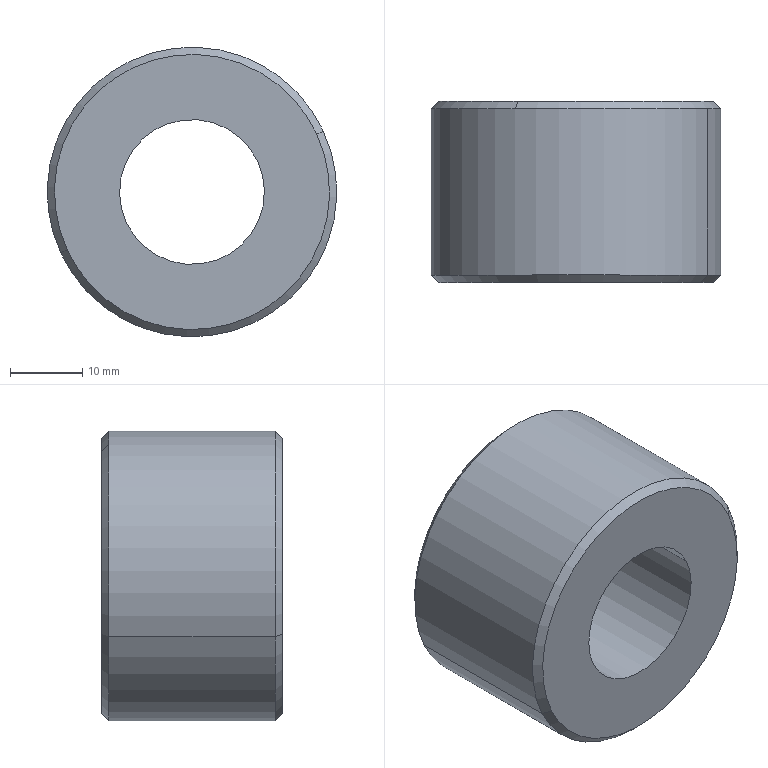Component | SolidWorks | RetainingRing-4 | 1 solid | 10 faces | box 40 x 25 x 40 mm | volume 23438 mm3 | cylinder 4 | cone 4 | plane 2 | commonest cylinder face diameters 20 x2 40 x2
STEP:
#1=CARTESIAN_POINT('',(-9.946,-3.568,-2.197));
#2=VERTEX_POINT('',#1);
#3=CARTESIAN_POINT('',(-10.661,-3.568,-2.528));
#4=VERTEX_POINT('',#3);
#5=CARTESIAN_POINT('',(-10.303,-3.568,-2.362));
#6=DIRECTION('',(-0.,1.,-0.));
#7=DIRECTION('',(-0.9074,0.,-0.4203));
#8=AXIS2_PLACEMENT_3D('',#5,#6,#7);
#9=CIRCLE('',#8,0.3937);
#10=EDGE_CURVE('',#2,#4,#9,.T.);
#11=ORIENTED_EDGE('',*,*,#10,.T.);
#12=CARTESIAN_POINT('',(-10.661,-4.552,-2.528));
#13=VERTEX_POINT('',#12);
#14=CARTESIAN_POINT('',(-10.661,-4.631,-2.528));
#15=DIRECTION('',(0.,-1.,0.));
#16=VECTOR('',#15,39.37);
#17=LINE('',#14,#16);
#18=EDGE_CURVE('',#4,#13,#17,.T.);
#19=ORIENTED_EDGE('',*,*,#18,.T.);
#20=CARTESIAN_POINT('',(-9.946,-4.552,-2.197));
#21=VERTEX_POINT('',#20);
#22=CARTESIAN_POINT('',(-10.303,-4.552,-2.362));
#23=DIRECTION('',(-0.,1.,-0.));
#24=DIRECTION('',(-0.9074,0.,-0.4203));
#25=AXIS2_PLACEMENT_3D('',#22,#23,#24);
#26=CIRCLE('',#25,0.3937);
#27=EDGE_CURVE('',#21,#13,#26,.T.);
#28=ORIENTED_EDGE('',*,*,#27,.F.);
#29=CARTESIAN_POINT('',(-9.946,-4.631,-2.197));
#30=DIRECTION('',(0.,-1.,0.));
#31=VECTOR('',#30,39.37);
#32=LINE('',#29,#31);
#33=EDGE_CURVE('',#2,#21,#32,.T.);
#34=ORIENTED_EDGE('',*,*,#33,.F.);
#35=EDGE_LOOP('',(#11,#19,#28,#34));
#36=FACE_OUTER_BOUND('',#35,.T.);
#37=CARTESIAN_POINT('',(-10.303,-4.631,-2.362));
#38=DIRECTION('',(0.,-1.,0.));
#39=DIRECTION('',(0.9074,0.,0.4203));
#40=AXIS2_PLACEMENT_3D('',#37,#38,#39);
#41=CYLINDRICAL_SURFACE('',#40,0.3937);
#42=ADVANCED_FACE('',(#36),#41,.F.);
#43=CARTESIAN_POINT('',(-10.634,-3.607,-1.648));
#44=VERTEX_POINT('',#43);
#45=CARTESIAN_POINT('',(-11.018,-3.607,-2.693));
#46=VERTEX_POINT('',#45);
#47=CARTESIAN_POINT('',(-10.303,-3.607,-2.362));
#48=DIRECTION('',(0.,-1.,0.));
#49=DIRECTION('',(0.9074,0.,0.4203));
#50=AXIS2_PLACEMENT_3D('',#47,#48,#49);
#51=CIRCLE('',#50,0.7874);
#52=EDGE_CURVE('',#44,#46,#51,.T.);
#53=ORIENTED_EDGE('',*,*,#52,.T.);
#54=CARTESIAN_POINT('',(-11.018,-4.513,-2.693));
#55=VERTEX_POINT('',#54);
#56=CARTESIAN_POINT('',(-11.018,-3.568,-2.693));
#57=DIRECTION('',(0.,-1.,0.));
#58=VECTOR('',#57,39.37);
#59=LINE('',#56,#58);
#60=EDGE_CURVE('',#46,#55,#59,.T.);
#61=ORIENTED_EDGE('',*,*,#60,.T.);
#62=CARTESIAN_POINT('',(-9.589,-4.513,-2.031));
#63=VERTEX_POINT('',#62);
#64=CARTESIAN_POINT('',(-10.303,-4.513,-2.362));
#65=DIRECTION('',(-0.,1.,-0.));
#66=DIRECTION('',(0.9074,0.,0.4203));
#67=AXIS2_PLACEMENT_3D('',#64,#65,#66);
#68=CIRCLE('',#67,0.7874);
#69=EDGE_CURVE('',#55,#63,#68,.T.);
#70=ORIENTED_EDGE('',*,*,#69,.T.);
#71=CARTESIAN_POINT('',(-9.589,-3.607,-2.031));
#72=VERTEX_POINT('',#71);
#73=CARTESIAN_POINT('',(-9.589,-3.568,-2.031));
#74=DIRECTION('',(0.,-1.,0.));
#75=VECTOR('',#74,39.37);
#76=LINE('',#73,#75);
#77=EDGE_CURVE('',#72,#63,#76,.T.);
#78=ORIENTED_EDGE('',*,*,#77,.F.);
#79=CARTESIAN_POINT('',(-10.303,-3.607,-2.362));
#80=DIRECTION('',(0.,-1.,0.));
#81=DIRECTION('',(0.9074,0.,0.4203));
#82=AXIS2_PLACEMENT_3D('',#79,#80,#81);
#83=CIRCLE('',#82,0.7874);
#84=EDGE_CURVE('',#72,#44,#83,.T.);
#85=ORIENTED_EDGE('',*,*,#84,.T.);
#86=EDGE_LOOP('',(#53,#61,#70,#78,#85));
#87=FACE_OUTER_BOUND('',#86,.T.);
#88=CARTESIAN_POINT('',(-10.303,-3.568,-2.362));
#89=DIRECTION('',(0.,-1.,0.));
#90=DIRECTION('',(0.9074,0.,0.4203));
#91=AXIS2_PLACEMENT_3D('',#88,#89,#90);
#92=CYLINDRICAL_SURFACE('',#91,0.7874);
#93=ADVANCED_FACE('',(#87),#92,.T.);
#94=CARTESIAN_POINT('',(-10.982,-4.552,-2.677));
#95=VERTEX_POINT('',#94);
#96=CARTESIAN_POINT('',(-9.625,-4.552,-2.048));
#97=VERTEX_POINT('',#96);
#98=CARTESIAN_POINT('',(-10.303,-4.552,-2.362));
#99=DIRECTION('',(-0.,1.,-0.));
#100=DIRECTION('',(-0.9074,0.,-0.4203));
#101=AXIS2_PLACEMENT_3D('',#98,#99,#100);
#102=CIRCLE('',#101,0.748);
#103=EDGE_CURVE('',#95,#97,#102,.T.);
#104=ORIENTED_EDGE('',*,*,#103,.T.);
#105=CARTESIAN_POINT('',(-9.589,-4.513,-2.031));
#106=DIRECTION('',(0.6416,0.7071,0.2972));
#107=VECTOR('',#106,39.37);
#108=LINE('',#105,#107);
#109=EDGE_CURVE('',#97,#63,#108,.T.);
#110=ORIENTED_EDGE('',*,*,#109,.T.);
#111=ORIENTED_EDGE('',*,*,#69,.F.);
#112=CARTESIAN_POINT('',(-11.018,-4.513,-2.693));
#113=DIRECTION('',(-0.6416,0.7071,-0.2972));
#114=VECTOR('',#113,39.37);
#115=LINE('',#112,#114);
#116=EDGE_CURVE('',#95,#55,#115,.T.);
#117=ORIENTED_EDGE('',*,*,#116,.F.);
#118=EDGE_LOOP('',(#104,#110,#111,#117));
#119=FACE_OUTER_BOUND('',#118,.T.);
#120=CARTESIAN_POINT('',(-10.303,-4.513,-2.362));
#121=DIRECTION('',(-0.,1.,-0.));
#122=DIRECTION('',(-0.9074,0.,-0.4203));
#123=AXIS2_PLACEMENT_3D('',#120,#121,#122);
#124=CONICAL_SURFACE('',#123,0.7874,0.7854);
#125=ADVANCED_FACE('',(#119),#124,.T.);
#126=CARTESIAN_POINT('',(-10.618,-3.568,-1.683));
#127=VERTEX_POINT('',#126);
#128=CARTESIAN_POINT('',(-9.989,-3.568,-3.041));
#129=VERTEX_POINT('',#128);
#130=CARTESIAN_POINT('',(-10.303,-3.568,-2.362));
#131=DIRECTION('',(0.,-1.,0.));
#132=DIRECTION('',(-0.4203,0.,0.9074));
#133=AXIS2_PLACEMENT_3D('',#130,#131,#132);
#134=CIRCLE('',#133,0.748);
#135=EDGE_CURVE('',#127,#129,#134,.T.);
#136=ORIENTED_EDGE('',*,*,#135,.T.);
#137=CARTESIAN_POINT('',(-9.972,-3.607,-3.077));
#138=VERTEX_POINT('',#137);
#139=CARTESIAN_POINT('',(-9.972,-3.607,-3.077));
#140=DIRECTION('',(0.2972,-0.7071,-0.6416));
#141=VECTOR('',#140,39.37);
#142=LINE('',#139,#141);
#143=EDGE_CURVE('',#129,#138,#142,.T.);
#144=ORIENTED_EDGE('',*,*,#143,.T.);
#145=CARTESIAN_POINT('',(-10.303,-3.607,-2.362));
#146=DIRECTION('',(0.,-1.,0.));
#147=DIRECTION('',(0.9074,0.,0.4203));
#148=AXIS2_PLACEMENT_3D('',#145,#146,#147);
#149=CIRCLE('',#148,0.7874);
#150=EDGE_CURVE('',#46,#138,#149,.T.);
#151=ORIENTED_EDGE('',*,*,#150,.F.);
#152=ORIENTED_EDGE('',*,*,#52,.F.);
#153=CARTESIAN_POINT('',(-10.634,-3.607,-1.648));
#154=DIRECTION('',(-0.2972,-0.7071,0.6416));
#155=VECTOR('',#154,39.37);
#156=LINE('',#153,#155);
#157=EDGE_CURVE('',#127,#44,#156,.T.);
#158=ORIENTED_EDGE('',*,*,#157,.F.);
#159=EDGE_LOOP('',(#136,#144,#151,#152,#158));
#160=FACE_OUTER_BOUND('',#159,.T.);
#161=CARTESIAN_POINT('',(-10.303,-3.607,-2.362));
#162=DIRECTION('',(0.,-1.,0.));
#163=DIRECTION('',(-0.4203,0.,0.9074));
#164=AXIS2_PLACEMENT_3D('',#161,#162,#163);
#165=CONICAL_SURFACE('',#164,0.7874,0.7854);
#166=ADVANCED_FACE('',(#160),#165,.T.);
#167=ORIENTED_EDGE('',*,*,#60,.F.);
#168=ORIENTED_EDGE('',*,*,#150,.T.);
#169=CARTESIAN_POINT('',(-10.303,-3.607,-2.362));
#170=DIRECTION('',(0.,-1.,0.));
#171=DIRECTION('',(0.9074,0.,0.4203));
#172=AXIS2_PLACEMENT_3D('',#169,#170,#171);
#173=CIRCLE('',#172,0.7874);
#174=EDGE_CURVE('',#138,#72,#173,.T.);
#175=ORIENTED_EDGE('',*,*,#174,.T.);
#176=ORIENTED_EDGE('',*,*,#77,.T.);
#177=CARTESIAN_POINT('',(-10.303,-4.513,-2.362));
#178=DIRECTION('',(-0.,1.,-0.));
#179=DIRECTION('',(0.9074,0.,0.4203));
#180=AXIS2_PLACEMENT_3D('',#177,#178,#179);
#181=CIRCLE('',#180,0.7874);
#182=EDGE_CURVE('',#63,#55,#181,.T.);
#183=ORIENTED_EDGE('',*,*,#182,.T.);
#184=EDGE_LOOP('',(#167,#168,#175,#176,#183));
#185=FACE_OUTER_BOUND('',#184,.T.);
#186=CARTESIAN_POINT('',(-10.303,-3.568,-2.362));
#187=DIRECTION('',(0.,-1.,0.));
#188=DIRECTION('',(0.9074,0.,0.4203));
#189=AXIS2_PLACEMENT_3D('',#186,#187,#188);
#190=CYLINDRICAL_SURFACE('',#189,0.7874);
#191=ADVANCED_FACE('',(#185),#190,.T.);
#192=ORIENTED_EDGE('',*,*,#109,.F.);
#193=CARTESIAN_POINT('',(-10.303,-4.552,-2.362));
#194=DIRECTION('',(-0.,1.,-0.));
#195=DIRECTION('',(-0.9074,0.,-0.4203));
#196=AXIS2_PLACEMENT_3D('',#193,#194,#195);
#197=CIRCLE('',#196,0.748);
#198=EDGE_CURVE('',#97,#95,#197,.T.);
#199=ORIENTED_EDGE('',*,*,#198,.T.);
#200=ORIENTED_EDGE('',*,*,#116,.T.);
#201=ORIENTED_EDGE('',*,*,#182,.F.);
#202=EDGE_LOOP('',(#192,#199,#200,#201));
#203=FACE_OUTER_BOUND('',#202,.T.);
#204=CARTESIAN_POINT('',(-10.303,-4.513,-2.362));
#205=DIRECTION('',(-0.,1.,-0.));
#206=DIRECTION('',(-0.9074,0.,-0.4203));
#207=AXIS2_PLACEMENT_3D('',#204,#205,#206);
#208=CONICAL_SURFACE('',#207,0.7874,0.7854);
#209=ADVANCED_FACE('',(#203),#208,.T.);
#210=ORIENTED_EDGE('',*,*,#143,.F.);
#211=CARTESIAN_POINT('',(-10.303,-3.568,-2.362));
#212=DIRECTION('',(0.,-1.,0.));
#213=DIRECTION('',(-0.4203,0.,0.9074));
#214=AXIS2_PLACEMENT_3D('',#211,#212,#213);
#215=CIRCLE('',#214,0.748);
#216=EDGE_CURVE('',#129,#127,#215,.T.);
#217=ORIENTED_EDGE('',*,*,#216,.T.);
#218=ORIENTED_EDGE('',*,*,#157,.T.);
#219=ORIENTED_EDGE('',*,*,#84,.F.);
#220=ORIENTED_EDGE('',*,*,#174,.F.);
#221=EDGE_LOOP('',(#210,#217,#218,#219,#220));
#222=FACE_OUTER_BOUND('',#221,.T.);
#223=CARTESIAN_POINT('',(-10.303,-3.607,-2.362));
#224=DIRECTION('',(0.,-1.,0.));
#225=DIRECTION('',(-0.4203,0.,0.9074));
#226=AXIS2_PLACEMENT_3D('',#223,#224,#225);
#227=CONICAL_SURFACE('',#226,0.7874,0.7854);
#228=ADVANCED_FACE('',(#222),#227,.T.);
#229=ORIENTED_EDGE('',*,*,#27,.T.);
#230=CARTESIAN_POINT('',(-10.303,-4.552,-2.362));
#231=DIRECTION('',(-0.,1.,-0.));
#232=DIRECTION('',(-0.9074,0.,-0.4203));
#233=AXIS2_PLACEMENT_3D('',#230,#231,#232);
#234=CIRCLE('',#233,0.3937);
#235=EDGE_CURVE('',#13,#21,#234,.T.);
#236=ORIENTED_EDGE('',*,*,#235,.T.);
#237=EDGE_LOOP('',(#229,#236));
#238=FACE_BOUND('',#237,.T.);
#239=ORIENTED_EDGE('',*,*,#103,.F.);
#240=ORIENTED_EDGE('',*,*,#198,.F.);
#241=EDGE_LOOP('',(#239,#240));
#242=FACE_OUTER_BOUND('',#241,.T.);
#243=CARTESIAN_POINT('',(-10.303,-4.552,-2.362));
#244=DIRECTION('',(-0.,1.,-0.));
#245=DIRECTION('',(-0.9074,-0.,-0.4203));
#246=AXIS2_PLACEMENT_3D('',#243,#244,#245);
#247=PLANE('',#246);
#248=ADVANCED_FACE('',(#238,#242),#247,.F.);
#249=ORIENTED_EDGE('',*,*,#10,.F.);
#250=CARTESIAN_POINT('',(-10.303,-3.568,-2.362));
#251=DIRECTION('',(-0.,1.,-0.));
#252=DIRECTION('',(-0.9074,0.,-0.4203));
#253=AXIS2_PLACEMENT_3D('',#250,#251,#252);
#254=CIRCLE('',#253,0.3937);
#255=EDGE_CURVE('',#4,#2,#254,.T.);
#256=ORIENTED_EDGE('',*,*,#255,.F.);
#257=EDGE_LOOP('',(#249,#256));
#258=FACE_BOUND('',#257,.T.);
#259=ORIENTED_EDGE('',*,*,#135,.F.);
#260=ORIENTED_EDGE('',*,*,#216,.F.);
#261=EDGE_LOOP('',(#259,#260));
#262=FACE_OUTER_BOUND('',#261,.T.);
#263=CARTESIAN_POINT('',(-10.303,-3.568,-2.362));
#264=DIRECTION('',(-0.,1.,-0.));
#265=DIRECTION('',(-0.9074,-0.,-0.4203));
#266=AXIS2_PLACEMENT_3D('',#263,#264,#265);
#267=PLANE('',#266);
#268=ADVANCED_FACE('',(#258,#262),#267,.T.);
#269=ORIENTED_EDGE('',*,*,#18,.F.);
#270=ORIENTED_EDGE('',*,*,#255,.T.);
#271=ORIENTED_EDGE('',*,*,#33,.T.);
#272=ORIENTED_EDGE('',*,*,#235,.F.);
#273=EDGE_LOOP('',(#269,#270,#271,#272));
#274=FACE_OUTER_BOUND('',#273,.T.);
#275=CARTESIAN_POINT('',(-10.303,-4.631,-2.362));
#276=DIRECTION('',(0.,-1.,0.));
#277=DIRECTION('',(0.9074,0.,0.4203));
#278=AXIS2_PLACEMENT_3D('',#275,#276,#277);
#279=CYLINDRICAL_SURFACE('',#278,0.3937);
#280=ADVANCED_FACE('',(#274),#279,.F.);
#281=CLOSED_SHELL('',(#42,#93,#125,#166,#191,#209,#228,#248,#268,#280));
#282=MANIFOLD_SOLID_BREP('',#281);
#283=CARTESIAN_POINT('',(0.,0.,0.));
#284=DIRECTION('',(0.,0.,1.));
#285=DIRECTION('',(1.,0.,0.));
#286=AXIS2_PLACEMENT_3D('',#283,#284,#285);
#287=(LENGTH_UNIT()NAMED_UNIT(*)SI_UNIT($,.METRE.));
#288=LENGTH_MEASURE_WITH_UNIT(LENGTH_MEASURE(0.0254),#287);
#289=DIMENSIONAL_EXPONENTS(1.,0.,0.,0.,0.,0.,0.);
#290=(CONVERSION_BASED_UNIT('',#288)LENGTH_UNIT()NAMED_UNIT(#289));
#291=UNCERTAINTY_MEASURE_WITH_UNIT(LENGTH_MEASURE(0.00001),#290,'','');
#292=(NAMED_UNIT(*)PLANE_ANGLE_UNIT()SI_UNIT($,.RADIAN.));
#293=(NAMED_UNIT(*)SI_UNIT($,.STERADIAN.)SOLID_ANGLE_UNIT());
#294=(GEOMETRIC_REPRESENTATION_CONTEXT(3)GLOBAL_UNCERTAINTY_ASSIGNED_CONTEXT((#291))GLOBAL_UNIT_ASSIGNED_CONTEXT((#290,#292,#293))REPRESENTATION_CONTEXT('',''));
#295=ADVANCED_BREP_SHAPE_REPRESENTATION('',(#282,#286),#294);
#296=COLOUR_RGB('',0.7922,0.8196,0.9333);
#297=FILL_AREA_STYLE_COLOUR('',#296);
#298=FILL_AREA_STYLE('',(#297));
#299=SURFACE_STYLE_FILL_AREA(#298);
#300=SURFACE_SIDE_STYLE('',(#299));
#301=SURFACE_STYLE_USAGE(.BOTH.,#300);
#302=PRESENTATION_STYLE_ASSIGNMENT((#301));
#303=STYLED_ITEM('',(#302),#282);
#304=(LENGTH_UNIT()NAMED_UNIT(*)SI_UNIT($,.METRE.));
#305=LENGTH_MEASURE_WITH_UNIT(LENGTH_MEASURE(0.0254),#304);
#306=DIMENSIONAL_EXPONENTS(1.,0.,0.,0.,0.,0.,0.);
#307=(CONVERSION_BASED_UNIT('',#305)LENGTH_UNIT()NAMED_UNIT(#306));
#308=UNCERTAINTY_MEASURE_WITH_UNIT(LENGTH_MEASURE(0.00001),#307,'','');
#309=(NAMED_UNIT(*)PLANE_ANGLE_UNIT()SI_UNIT($,.RADIAN.));
#310=(NAMED_UNIT(*)SI_UNIT($,.STERADIAN.)SOLID_ANGLE_UNIT());
#311=(GEOMETRIC_REPRESENTATION_CONTEXT(3)GLOBAL_UNCERTAINTY_ASSIGNED_CONTEXT((#308))GLOBAL_UNIT_ASSIGNED_CONTEXT((#307,#309,#310))REPRESENTATION_CONTEXT('',''));
#312=MECHANICAL_DESIGN_GEOMETRIC_PRESENTATION_REPRESENTATION('',(#303),#311);
#313=PRESENTATION_LAYER_ASSIGNMENT('','',(#303));